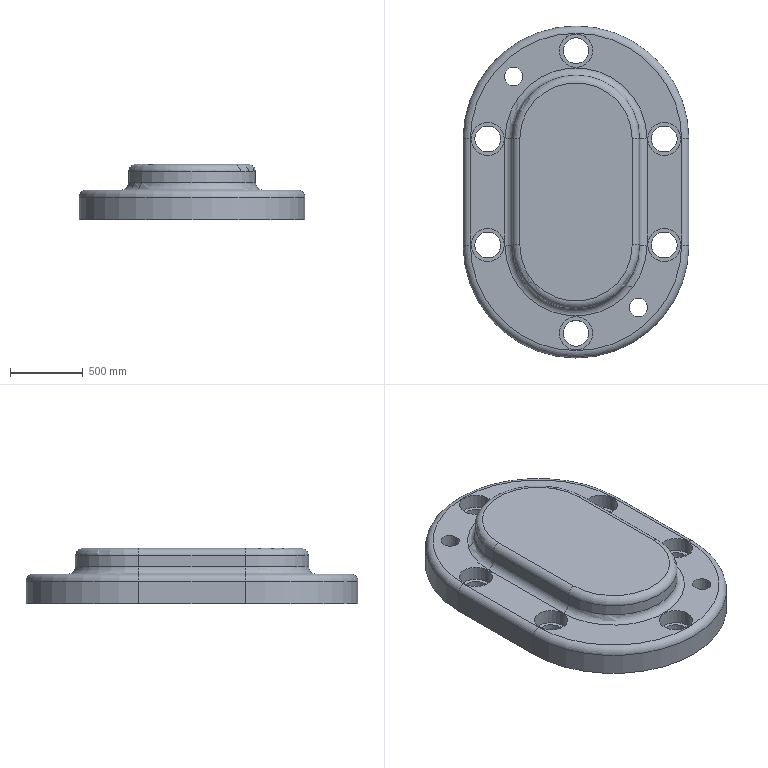Component | NX | 1 | 1 solid | 47 faces | volume 713348545 mm3 | cylinder 26 | plane 13 | torus 6 | cone 2 | commonest cylinder face diameters 177.8 x6 101.6 x6 228.6 x6 1555.496 x2 876.3 x2 127 x2 406.4 x2